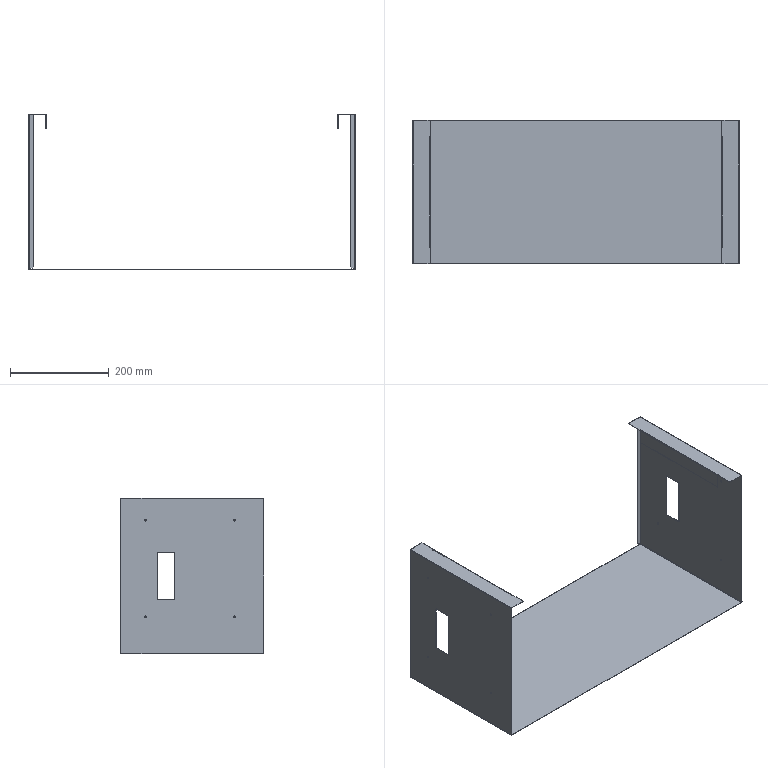Component | SolidWorks | PC-CAJ-P09-1_PM-CAJ-P37-1 | 1 solid | 120 faces | volume 283333 mm3 | plane 88 | cylinder 32 | commonest cylinder face diameters 3 x16 1 x8 2.4 x8 | material Plain Carbon Steel